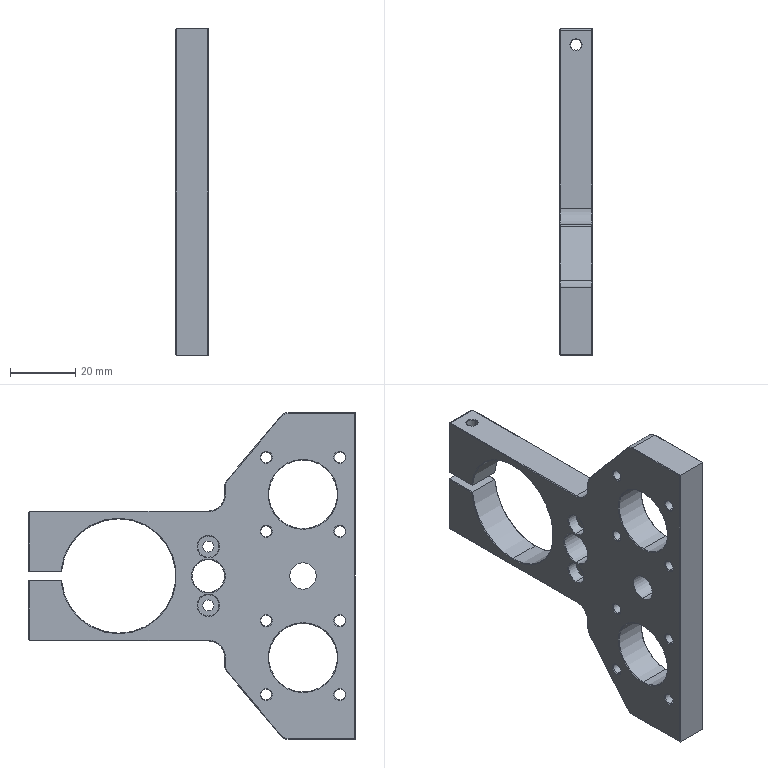Component | SolidWorks | Z-AxisElectricScrewdriverFixingPlate-1 | 1 solid | 171 faces | box 10 x 100 x 100 mm | volume 40294 mm3 | cylinder 62 | cone 41 | torus 37 | plane 31 | commonest cylinder face diameters 3.3 x18 0.4 x13 6.5 x4 3.4 x4 10 x4 21 x4 6 x4 35 x3
build123d program:
from build123d import *

# Parameters (mm, degrees)
BOSS_EXTRUDE1_DEPTH                             = 10
SKETCH2_W                                       = 39.76
SKETCH2_H                                       = 10
BOSS_EXTRUDE2_DEPTH                             = 60
CUT_EXTRUDE1_DEPTH                              = 142.774
SKETCH4_W                                       = 17.5
SKETCH4_H                                       = 10
F_4_7_4_7_DIAMETER_HOLE1_D                      = 4.7
M4_TAPPED_HOLE1_D                               = 3.3
F_21_0_21_DIAMETER_HOLE1_D                      = 21
M4_HEX_SOCKET_HEAD_CAP_SCREW_CBORE1_D           = 4.8
M4_HEX_SOCKET_HEAD_CAP_SCREW_CBORE1_DEPTH       = 18.63
M4_HEX_SOCKET_HEAD_CAP_SCREW_CBORE1_CBORE_D     = 8
M4_HEX_SOCKET_HEAD_CAP_SCREW_CBORE1_CBORE_DEPTH = 4.4
M4_TAPPED_HOLE2_D                               = 3.3
FILLET1_R                                       = 5
SKETCH15_R                                      = 5
CUT_EXTRUDE2_DEPTH                              = 142.774
M3_HEX_SOCKET_HEAD_CAP_SCREW_CBORE1_D           = 3.4
M3_HEX_SOCKET_HEAD_CAP_SCREW_CBORE1_CBORE_D     = 6.5
M3_HEX_SOCKET_HEAD_CAP_SCREW_CBORE1_CBORE_DEPTH = 3.4
FILLET2_R                                       = 3
FILLET3_R                                       = 0.5
CHAMFER1_SIZE                                   = 0.2
FILLET4_R                                       = 0.2
CHAMFER2_SIZE                                   = 0.2
F_8_1_8_1_DIAMETER_HOLE1_D                      = 8.1
F_8_1_8_1_DIAMETER_HOLE1_DEPTH                  = 10


with BuildPart() as part:
    # Sketch1 → Boss-Extrude1 (new body)
    with BuildSketch(Plane(origin=(0, 0, -10), x_dir=(-1, 0, 0), z_dir=(0, 0, -1))):
        Polygon((0, 22), (-21.5, 40), (-78.5, 40), (-100, 22), (-100, 0), (0, 0), align=None)
    extrude(amount=-BOSS_EXTRUDE1_DEPTH)

    # Sketch2 → Boss-Extrude2 (add)
    with BuildSketch(Plane(origin=(0, 40, 0), x_dir=(-1, 0, 0), z_dir=(0, 1, 0))):
        with Locations((-50, -5)):
            Rectangle(SKETCH2_W, SKETCH2_H)
    extrude(amount=BOSS_EXTRUDE2_DEPTH)

    # Sketch3 → Cut-Extrude1 (cut, through all)
    with BuildSketch(Plane.XY):
        with BuildLine():
            Line((48.75, 100), (48.75, 89.955))
            ThreePointArc((48.75, 89.955), (50, 90), (51.25, 89.955))
            Line((51.25, 89.955), (51.25, 100))
            Line((51.25, 100), (48.75, 100))
        make_face()
    extrude(amount=-CUT_EXTRUDE1_DEPTH, mode=Mode.SUBTRACT)

    # Sketch4 → Cut-Revolve1 (revolve, cut)
    with BuildSketch(Plane(origin=(0, 72.5, 0), x_dir=(1, 0, 0), z_dir=(0, 1, 0))):
        with Locations((58.75, 5)):
            Rectangle(SKETCH4_W, SKETCH4_H)
    revolve(axis=Axis((50, 72.5, -10), (0, 0, 1)), mode=Mode.SUBTRACT)

    # 4.7 _4.7_ Diameter Hole1 (through all)
    with Locations(Plane(origin=(0, 0, -10), x_dir=(-1, 0, 0), z_dir=(0, 0, -1))):
        with Locations((-50, 15.5), (-50, 45)):
            Hole(F_4_7_4_7_DIAMETER_HOLE1_D / 2)

    # M4 Tapped Hole1 (through all)
    with Locations(Plane(origin=(0, 0, -10), x_dir=(-1, 0, 0), z_dir=(0, 0, -1))):
        with Locations((-13.69, 27.31), (-36.31, 27.31), (-36.31, 4.69), (-13.69, 4.69), (-63.69, 27.31), (-86.31, 27.31), (-86.31, 4.69), (-63.69, 4.69)):
            Hole(M4_TAPPED_HOLE1_D / 2)

    # 21.0 _21_ Diameter Hole1 (through all)
    with Locations(Plane(origin=(0, 0, -10), x_dir=(-1, 0, 0), z_dir=(0, 0, -1))):
        with Locations((-25, 16), (-75, 16)):
            Hole(F_21_0_21_DIAMETER_HOLE1_D / 2)

    # M4 Hex Socket Head Cap Screw CBORE1
    with Locations(Plane(origin=(69.88, 0, 0), x_dir=(0, 0, -1), z_dir=(1, 0, 0))):
        with Locations((5, 95)):
            CounterBoreHole(M4_HEX_SOCKET_HEAD_CAP_SCREW_CBORE1_D / 2, M4_HEX_SOCKET_HEAD_CAP_SCREW_CBORE1_CBORE_D / 2, M4_HEX_SOCKET_HEAD_CAP_SCREW_CBORE1_CBORE_DEPTH, depth=M4_HEX_SOCKET_HEAD_CAP_SCREW_CBORE1_DEPTH)

    # M4 Tapped Hole2 (through all)
    with Locations(Plane(origin=(48.75, 0, 0), x_dir=(0, 0, -1), z_dir=(1, 0, 0))):
        with Locations((5, 95)):
            Hole(M4_TAPPED_HOLE2_D / 2)

    # Fillet1
    fillet1_edges = [part.edges().sort_by_distance(p)[0] for p in [
        (69.88, 40, -5),
        (30.12, 40, -5),
    ]]
    fillet(fillet1_edges, radius=FILLET1_R)

    # Sketch15 → Cut-Extrude2 (cut, through all)
    with BuildSketch(Plane(origin=(0, 0, -10), x_dir=(-1, 0, 0), z_dir=(0, 0, -1))):
        with Locations((-50, 45)):
            Circle(SKETCH15_R)
    extrude(amount=-CUT_EXTRUDE2_DEPTH, mode=Mode.SUBTRACT)

    # M3 Hex Socket Head Cap Screw CBORE1 (through all)
    with Locations(Plane(origin=(0, 0, -10), x_dir=(-1, 0, 0), z_dir=(0, 0, -1))):
        with Locations((-59, 45), (-41, 45)):
            CounterBoreHole(M3_HEX_SOCKET_HEAD_CAP_SCREW_CBORE1_D / 2, M3_HEX_SOCKET_HEAD_CAP_SCREW_CBORE1_CBORE_D / 2, M3_HEX_SOCKET_HEAD_CAP_SCREW_CBORE1_CBORE_DEPTH)

    # Fillet2
    fillet2_edges = [part.edges().sort_by_distance(p)[0] for p in [
        (100, 22, -5),
        (78.5, 40, -5),
        (21.5, 40, -5),
        (0, 22, -5),
    ]]
    fillet(fillet2_edges, radius=FILLET2_R)

    # Fillet3
    fillet3_edges = [part.edges().sort_by_distance(p)[0] for p in [
        (69.88, 100, -5),
        (30.12, 100, -5),
    ]]
    fillet(fillet3_edges, radius=FILLET3_R)

    # Chamfer1
    chamfer1_edges = [part.edges().sort_by_distance(p)[0] for p in [
        (34.66, 4.69, -10),
        (34.66, 27.31, -10),
        (12.04, 27.31, -10),
        (64.5, 16, -10),
        (14.5, 16, -10),
        (76.145, 40, -10),
        (71.344, 41.464, -10),
        (28.656, 41.464, -10),
        (55, 45, -10),
        (44.25, 45, -10),
        (62.25, 45, -10),
        (89.131, 31.1, -10),
        (100, 10.3, -10),
        (10.869, 31.1, -10),
        (23.855, 40, -10),
        (0.2818, 21.868, -10),
        (21.566, 39.82, -10),
        (78.434, 39.82, -10),
        (99.718, 21.868, -10),
        (60.315, 100, -10),
        (30.12, 72.25, -10),
        (69.88, 72.25, -10),
        (30.266, 99.854, -10),
        (69.734, 99.854, -10),
        (39.685, 100, -10),
        (51.25, 94.978, -10),
        (48.75, 94.978, -10),
        (38.076, 59.691, -10),
        (50, 0, -10),
        (47.65, 15.5, -10),
        (62.04, 4.69, -10),
        (84.66, 4.69, -10),
        (0, 10.3, -10),
        (84.66, 27.31, -10),
        (62.04, 27.31, -10),
        (12.04, 4.69, -10),
    ]]
    chamfer(chamfer1_edges, length=CHAMFER1_SIZE)

    # Fillet4
    fillet4_edges = [part.edges().sort_by_distance(p)[0] for p in [
        (34.66, 4.69, 0),
        (34.66, 27.31, 0),
        (12.04, 27.31, 0),
        (64.5, 16, 0),
        (14.5, 16, 0),
        (76.145, 40, 0),
        (71.344, 41.464, 0),
        (28.656, 41.464, 0),
        (55, 45, 0),
        (39.3, 45, 0),
        (57.3, 45, 0),
        (89.131, 31.1, 0),
        (50, 0, 0),
        (100, 10.3, 0),
        (23.855, 40, 0),
        (10.869, 31.1, 0),
        (0.2818, 21.868, 0),
        (21.566, 39.82, 0),
        (78.434, 39.82, 0),
        (99.718, 21.868, 0),
        (69.88, 72.25, 0),
        (39.685, 100, 0),
        (30.12, 72.25, 0),
        (30.266, 99.854, 0),
        (69.734, 99.854, 0),
        (60.315, 100, 0),
        (0, 10.3, 0),
        (48.75, 94.978, 0),
        (51.25, 94.978, 0),
        (38.076, 59.691, 0),
        (47.65, 15.5, 0),
        (62.04, 4.69, 0),
        (84.66, 4.69, 0),
        (84.66, 27.31, 0),
        (62.04, 27.31, 0),
        (12.04, 4.69, 0),
    ]]
    fillet(fillet4_edges, radius=FILLET4_R)

    # Chamfer2
    chamfer2_edges = [part.edges().sort_by_distance(p)[0] for p in [
        (69.88, 95, -1),
        (30.12, 95, -6.65),
    ]]
    chamfer(chamfer2_edges, length=CHAMFER2_SIZE)

    # 8.1 _8.1_ Diameter Hole1
    with Locations(Plane.XY):
        with Locations((50, 16)):
            Hole(F_8_1_8_1_DIAMETER_HOLE1_D / 2, depth=F_8_1_8_1_DIAMETER_HOLE1_DEPTH)


solid = part.part

# Placed as in the assembly
solid = solid.moved(Location((-68.981, 52.516, 132), (0, 90, 0)))